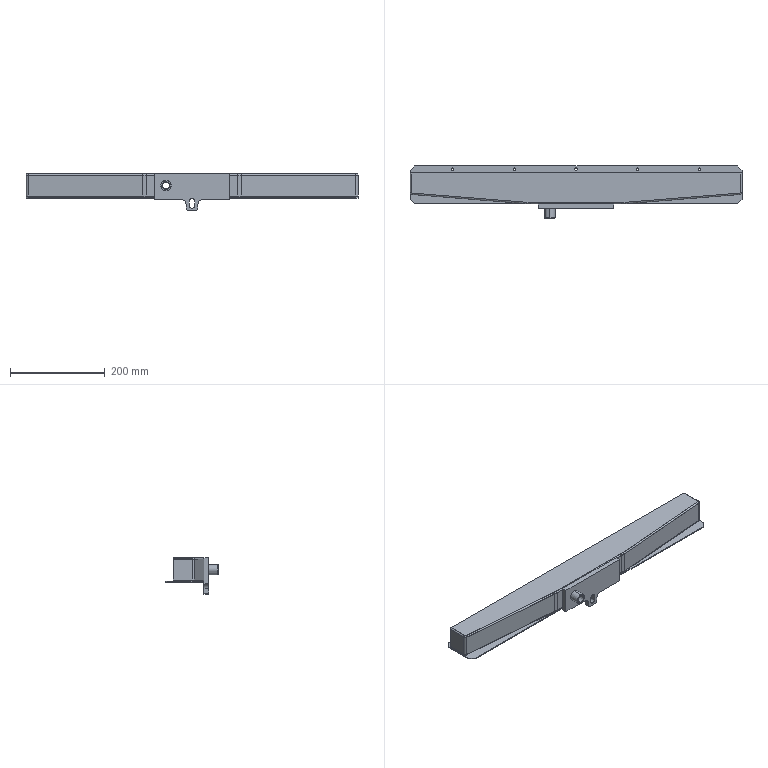Component | SolidWorks | AUTO-SpinDryWashing-01-03000002-1 | 4 solids | 117 faces | volume 313085 mm3 | plane 46 | cylinder 41 | torus 16 | cone 14 | commonest cylinder face diameters 6 x10 4 x10 22 x6 11 x3 20 x2 14.3 x2 200 x2 10 x2 | material AISI 316 Stainless Steel Sheet (SS)